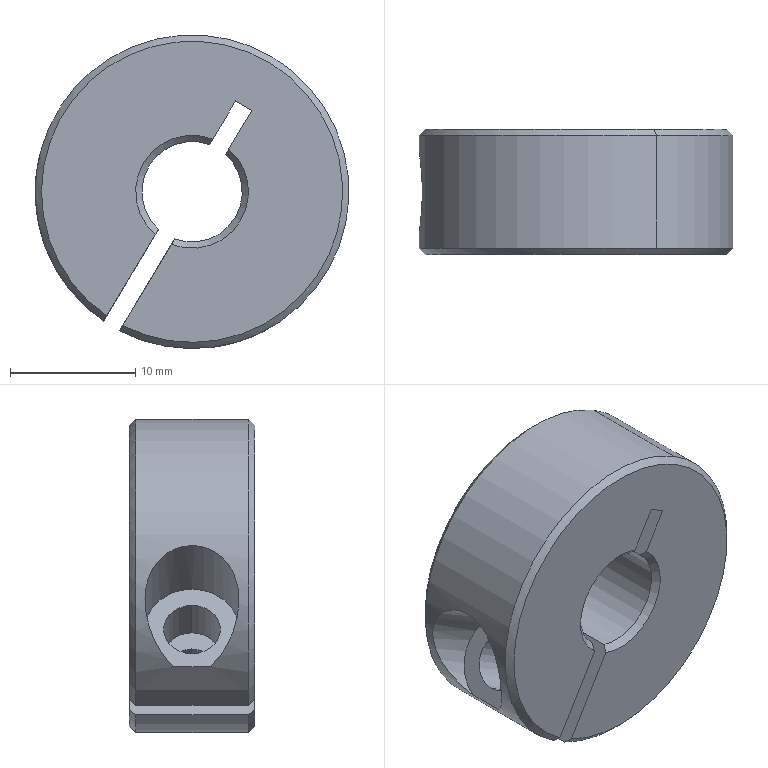Component | SolidWorks | F12529-M1072-1 | 1 solid | 24 faces | box 25 x 10 x 25 mm | volume 3862 mm3 | cylinder 9 | plane 8 | cone 7 | commonest cylinder face diameters 3.3 x2 4.5 x2 25 x2 8 x2 7.5 x1
build123d program:
from build123d import *

# Parameters (mm, degrees)
SKETCH1_R           = 12.5
SKETCH1_R_2         = 4
BOSS_EXTRUDE1_DEPTH = 10
CHAMFER1_SIZE       = 0.5
SKETCH2_W           = 1.5
SKETCH2_H           = 21
CUT_EXTRUDE1_DEPTH  = 12
SKETCH5_R           = 3.75
CUT_EXTRUDE2_DEPTH  = 10
SKETCH6_R           = 2.25
CUT_EXTRUDE3_DEPTH  = 5
M4_TAPPED_HOLE1_D   = 3.3


with BuildPart() as part:
    # Sketch1 → Boss-Extrude1 (new body)
    with BuildSketch(Plane(origin=(0, 0, 0), x_dir=(1, 0, 0), z_dir=(0, 1, 0))):
        with Locations(Location((0, 0, 0), (0, 0, 270))):
            Circle(SKETCH1_R)
        with Locations(Location((0, 0, 0), (0, 0, 270))):
            Circle(SKETCH1_R_2, mode=Mode.SUBTRACT)
    extrude(amount=BOSS_EXTRUDE1_DEPTH)

    # Chamfer1
    chamfer1_edges = [part.edges().sort_by_distance(p)[0] for p in [
        (0, 0, -12.5),
        (0, 10, -12.5),
        (0, 0, -4),
        (0, 10, -4),
    ]]
    chamfer(chamfer1_edges, length=CHAMFER1_SIZE)

    # Sketch2 → Cut-Extrude1 (cut)
    with BuildSketch(Plane(origin=(0, 10, 0), x_dir=(1, 0, 0), z_dir=(0, 1, 0))):
        with Locations((0, -2.5)):
            Rectangle(SKETCH2_W, SKETCH2_H)
    extrude(amount=-CUT_EXTRUDE1_DEPTH, mode=Mode.SUBTRACT)

    # Sketch5 → Cut-Extrude2 (cut)
    with BuildSketch(Plane(origin=(5, 0, 0), x_dir=(0, 0, -1), z_dir=(1, 0, 0))):
        with Locations((-8, 5)):
            Circle(SKETCH5_R)
    extrude(amount=CUT_EXTRUDE2_DEPTH, mode=Mode.SUBTRACT)

    # Sketch6 → Cut-Extrude3 (cut)
    with BuildSketch(Plane(origin=(5, 0, 0), x_dir=(0, 0, -1), z_dir=(1, 0, 0))):
        with Locations((-8, 5)):
            Circle(SKETCH6_R)
    extrude(amount=-CUT_EXTRUDE3_DEPTH, mode=Mode.SUBTRACT)

    # M4 Tapped Hole1 (through all)
    with Locations(Plane(origin=(-0.75, 0, 0), x_dir=(0, 0, -1), z_dir=(1, 0, 0))):
        with Locations((-8, 5)):
            Hole(M4_TAPPED_HOLE1_D / 2)


solid = part.part

# Placed as in the assembly
solid = solid.moved(Location((37.5, -20, 20), (179.999, -31.002, -179.999)))
STEP:
#1=COLOUR_RGB('',0.7922,0.8196,0.9333);
#2=FILL_AREA_STYLE_COLOUR('',#1);
#3=FILL_AREA_STYLE('',(#2));
#4=SURFACE_STYLE_FILL_AREA(#3);
#5=SURFACE_SIDE_STYLE('',(#4));
#6=SURFACE_STYLE_USAGE(.BOTH.,#5);
#7=PRESENTATION_STYLE_ASSIGNMENT((#6));
#8=CARTESIAN_POINT('',(1.549,-0.5906,0.3006));
#9=VERTEX_POINT('',#8);
#10=CARTESIAN_POINT('',(1.711,-0.5906,0.3548));
#11=VERTEX_POINT('',#10);
#12=CARTESIAN_POINT('',(1.549,-0.5906,0.3006));
#13=CARTESIAN_POINT('',(1.549,-0.5955,0.3006));
#14=CARTESIAN_POINT('',(1.55,-0.6005,0.3008));
#15=CARTESIAN_POINT('',(1.553,-0.6099,0.3013));
#16=CARTESIAN_POINT('',(1.555,-0.6143,0.3017));
#17=CARTESIAN_POINT('',(1.564,-0.6263,0.3031));
#18=CARTESIAN_POINT('',(1.572,-0.6329,0.3045));
#19=CARTESIAN_POINT('',(1.588,-0.6435,0.308));
#20=CARTESIAN_POINT('',(1.597,-0.6475,0.3102));
#21=CARTESIAN_POINT('',(1.615,-0.6533,0.3151));
#22=CARTESIAN_POINT('',(1.625,-0.655,0.318));
#23=CARTESIAN_POINT('',(1.643,-0.6558,0.3243));
#24=CARTESIAN_POINT('',(1.652,-0.655,0.3278));
#25=CARTESIAN_POINT('',(1.666,-0.6514,0.3332));
#26=CARTESIAN_POINT('',(1.67,-0.6498,0.335));
#27=CARTESIAN_POINT('',(1.678,-0.6458,0.3387));
#28=CARTESIAN_POINT('',(1.682,-0.6434,0.3405));
#29=CARTESIAN_POINT('',(1.694,-0.6349,0.3457));
#30=CARTESIAN_POINT('',(1.7,-0.6278,0.3489));
#31=CARTESIAN_POINT('',(1.706,-0.6147,0.3523));
#32=CARTESIAN_POINT('',(1.708,-0.6101,0.3532));
#33=CARTESIAN_POINT('',(1.71,-0.6006,0.3544));
#34=CARTESIAN_POINT('',(1.711,-0.5956,0.3548));
#35=CARTESIAN_POINT('',(1.711,-0.5906,0.3548));
#36=B_SPLINE_CURVE_WITH_KNOTS('',3,(#12,#13,#14,#15,#16,#17,#18,#19,#20,#21,#22,#23,#24,#25,#26,#27,#28,#29,#30,#31,#32,#33,#34,#35),.UNSPECIFIED.,.F.,.F.,(4,2,2,2,2,2,2,2,2,2,2,4),(0.006013,0.006389,0.006765,0.007517,0.008269,0.009021,0.009773,0.01015,0.01053,0.01128,0.01165,0.01203),.UNSPECIFIED.);
#37=EDGE_CURVE('',#9,#11,#36,.T.);
#38=ORIENTED_EDGE('',*,*,#37,.F.);
#39=CARTESIAN_POINT('',(1.306,-0.5906,0.4465));
#40=VERTEX_POINT('',#39);
#41=CARTESIAN_POINT('',(1.306,-0.5906,0.4465));
#42=DIRECTION('',(-0.8571,0.,0.5151));
#43=VECTOR('',#42,39.37);
#44=LINE('',#41,#43);
#45=EDGE_CURVE('',#9,#40,#44,.T.);
#46=ORIENTED_EDGE('',*,*,#45,.T.);
#47=CARTESIAN_POINT('',(1.373,-0.5906,0.5579));
#48=VERTEX_POINT('',#47);
#49=CARTESIAN_POINT('',(1.339,-0.5906,0.5022));
#50=DIRECTION('',(-0.8571,0.,0.5151));
#51=DIRECTION('',(0.5151,0.,0.8571));
#52=AXIS2_PLACEMENT_3D('',#49,#50,#51);
#53=CIRCLE('',#52,0.06496);
#54=EDGE_CURVE('',#40,#48,#53,.T.);
#55=ORIENTED_EDGE('',*,*,#54,.T.);
#56=CARTESIAN_POINT('',(1.373,-0.5906,0.5579));
#57=DIRECTION('',(-0.8571,0.,0.5151));
#58=VECTOR('',#57,39.37);
#59=LINE('',#56,#58);
#60=EDGE_CURVE('',#11,#48,#59,.T.);
#61=ORIENTED_EDGE('',*,*,#60,.F.);
#62=EDGE_LOOP('',(#38,#46,#55,#61));
#63=FACE_OUTER_BOUND('',#62,.T.);
#64=CARTESIAN_POINT('',(1.339,-0.5906,0.5022));
#65=DIRECTION('',(-0.8571,0.,0.5151));
#66=DIRECTION('',(0.5151,0.,0.8571));
#67=AXIS2_PLACEMENT_3D('',#64,#65,#66);
#68=CYLINDRICAL_SURFACE('',#67,0.06496);
#69=ADVANCED_FACE('',(#63),#68,.F.);
#70=CARTESIAN_POINT('',(1.243,-0.5906,0.4567));
#71=VERTEX_POINT('',#70);
#72=CARTESIAN_POINT('',(1.334,-0.5906,0.6086));
#73=VERTEX_POINT('',#72);
#74=CARTESIAN_POINT('',(1.289,-0.5906,0.5326));
#75=DIRECTION('',(-0.8571,0.,0.5151));
#76=DIRECTION('',(0.5151,0.,0.8571));
#77=AXIS2_PLACEMENT_3D('',#74,#75,#76);
#78=CIRCLE('',#77,0.08858);
#79=EDGE_CURVE('',#71,#73,#78,.T.);
#80=ORIENTED_EDGE('',*,*,#79,.F.);
#81=CARTESIAN_POINT('',(1.1,-0.5906,0.5429));
#82=VERTEX_POINT('',#81);
#83=CARTESIAN_POINT('',(1.269,-0.5906,0.4415));
#84=DIRECTION('',(-0.8571,0.,0.5151));
#85=VECTOR('',#84,39.37);
#86=LINE('',#83,#85);
#87=EDGE_CURVE('',#71,#82,#86,.T.);
#88=ORIENTED_EDGE('',*,*,#87,.T.);
#89=CARTESIAN_POINT('',(1.191,-0.5906,0.6948));
#90=VERTEX_POINT('',#89);
#91=CARTESIAN_POINT('',(1.145,-0.5906,0.6188));
#92=DIRECTION('',(-0.8571,0.,0.5151));
#93=DIRECTION('',(0.5151,0.,0.8571));
#94=AXIS2_PLACEMENT_3D('',#91,#92,#93);
#95=CIRCLE('',#94,0.08858);
#96=EDGE_CURVE('',#82,#90,#95,.T.);
#97=ORIENTED_EDGE('',*,*,#96,.T.);
#98=CARTESIAN_POINT('',(1.36,-0.5906,0.5934));
#99=DIRECTION('',(-0.8571,0.,0.5151));
#100=VECTOR('',#99,39.37);
#101=LINE('',#98,#100);
#102=EDGE_CURVE('',#73,#90,#101,.T.);
#103=ORIENTED_EDGE('',*,*,#102,.F.);
#104=EDGE_LOOP('',(#80,#88,#97,#103));
#105=FACE_OUTER_BOUND('',#104,.T.);
#106=CARTESIAN_POINT('',(1.314,-0.5906,0.5174));
#107=DIRECTION('',(-0.8571,0.,0.5151));
#108=DIRECTION('',(0.5151,0.,0.8571));
#109=AXIS2_PLACEMENT_3D('',#106,#107,#108);
#110=CYLINDRICAL_SURFACE('',#109,0.08858);
#111=ADVANCED_FACE('',(#105),#110,.F.);
#112=CARTESIAN_POINT('',(1.72,-0.3937,1.192));
#113=VERTEX_POINT('',#112);
#114=CARTESIAN_POINT('',(1.259,-0.3937,0.368));
#115=VERTEX_POINT('',#114);
#116=CARTESIAN_POINT('',(1.476,-0.3937,0.7874));
#117=DIRECTION('',(0.,1.,0.));
#118=DIRECTION('',(-0.5151,0.,-0.8571));
#119=AXIS2_PLACEMENT_3D('',#116,#117,#118);
#120=CIRCLE('',#119,0.4724);
#121=EDGE_CURVE('',#113,#115,#120,.T.);
#122=ORIENTED_EDGE('',*,*,#121,.F.);
#123=CARTESIAN_POINT('',(1.73,-0.4134,1.209));
#124=VERTEX_POINT('',#123);
#125=CARTESIAN_POINT('',(1.72,-0.3937,1.192));
#126=DIRECTION('',(0.3642,-0.7071,0.6061));
#127=VECTOR('',#126,39.37);
#128=LINE('',#125,#127);
#129=EDGE_CURVE('',#113,#124,#128,.T.);
#130=ORIENTED_EDGE('',*,*,#129,.T.);
#131=CARTESIAN_POINT('',(1.249,-0.4134,0.3511));
#132=VERTEX_POINT('',#131);
#133=CARTESIAN_POINT('',(1.476,-0.4134,0.7874));
#134=DIRECTION('',(0.,-1.,0.));
#135=DIRECTION('',(-0.5151,0.,-0.8571));
#136=AXIS2_PLACEMENT_3D('',#133,#134,#135);
#137=CIRCLE('',#136,0.4921);
#138=EDGE_CURVE('',#132,#124,#137,.T.);
#139=ORIENTED_EDGE('',*,*,#138,.F.);
#140=CARTESIAN_POINT('',(1.259,-0.3937,0.368));
#141=CARTESIAN_POINT('',(1.255,-0.4003,0.3624));
#142=CARTESIAN_POINT('',(1.252,-0.4068,0.3568));
#143=CARTESIAN_POINT('',(1.249,-0.4134,0.3511));
#144=B_SPLINE_CURVE_WITH_KNOTS('',3,(#140,#141,#142,#143),.UNSPECIFIED.,.F.,.F.,(4,4),(0.04478,0.04549),.UNSPECIFIED.);
#145=EDGE_CURVE('',#115,#132,#144,.T.);
#146=ORIENTED_EDGE('',*,*,#145,.F.);
#147=EDGE_LOOP('',(#122,#130,#139,#146));
#148=FACE_OUTER_BOUND('',#147,.T.);
#149=CARTESIAN_POINT('',(1.476,-0.3937,0.7874));
#150=DIRECTION('',(0.,-1.,0.));
#151=DIRECTION('',(0.5151,0.,0.8571));
#152=AXIS2_PLACEMENT_3D('',#149,#150,#151);
#153=CONICAL_SURFACE('',#152,0.4724,0.7854);
#154=ADVANCED_FACE('',(#148),#153,.T.);
#155=CARTESIAN_POINT('',(1.711,-0.5906,0.3548));
#156=CARTESIAN_POINT('',(1.711,-0.5855,0.3548));
#157=CARTESIAN_POINT('',(1.71,-0.5807,0.3545));
#158=CARTESIAN_POINT('',(1.708,-0.5711,0.3532));
#159=CARTESIAN_POINT('',(1.706,-0.5664,0.3523));
#160=CARTESIAN_POINT('',(1.702,-0.5579,0.3501));
#161=CARTESIAN_POINT('',(1.699,-0.5538,0.3487));
#162=CARTESIAN_POINT('',(1.693,-0.5466,0.3456));
#163=CARTESIAN_POINT('',(1.69,-0.5434,0.344));
#164=CARTESIAN_POINT('',(1.682,-0.5377,0.3405));
#165=CARTESIAN_POINT('',(1.679,-0.5353,0.3387));
#166=CARTESIAN_POINT('',(1.67,-0.5314,0.335));
#167=CARTESIAN_POINT('',(1.666,-0.5298,0.3332));
#168=CARTESIAN_POINT('',(1.653,-0.5262,0.3278));
#169=CARTESIAN_POINT('',(1.643,-0.5253,0.3243));
#170=CARTESIAN_POINT('',(1.624,-0.5261,0.318));
#171=CARTESIAN_POINT('',(1.615,-0.5278,0.3151));
#172=CARTESIAN_POINT('',(1.597,-0.5336,0.3101));
#173=CARTESIAN_POINT('',(1.588,-0.5376,0.308));
#174=CARTESIAN_POINT('',(1.576,-0.5456,0.3054));
#175=CARTESIAN_POINT('',(1.572,-0.5485,0.3046));
#176=CARTESIAN_POINT('',(1.565,-0.5551,0.3032));
#177=CARTESIAN_POINT('',(1.561,-0.5588,0.3026));
#178=CARTESIAN_POINT('',(1.555,-0.5669,0.3017));
#179=CARTESIAN_POINT('',(1.553,-0.5712,0.3013));
#180=CARTESIAN_POINT('',(1.55,-0.5806,0.3008));
#181=CARTESIAN_POINT('',(1.549,-0.5856,0.3006));
#182=CARTESIAN_POINT('',(1.549,-0.5906,0.3006));
#183=B_SPLINE_CURVE_WITH_KNOTS('',3,(#155,#156,#157,#158,#159,#160,#161,#162,#163,#164,#165,#166,#167,#168,#169,#170,#171,#172,#173,#174,#175,#176,#177,#178,#179,#180,#181,#182),.UNSPECIFIED.,.F.,.F.,(4,2,2,2,2,2,2,2,2,2,2,2,2,4),(0.,0.0003758,0.0007516,0.001127,0.001503,0.001879,0.002255,0.003006,0.003758,0.004509,0.004885,0.005261,0.005637,0.006013),.UNSPECIFIED.);
#184=EDGE_CURVE('',#11,#9,#183,.T.);
#185=ORIENTED_EDGE('',*,*,#184,.T.);
#186=ORIENTED_EDGE('',*,*,#37,.T.);
#187=EDGE_LOOP('',(#185,#186));
#188=FACE_BOUND('',#187,.T.);
#189=ORIENTED_EDGE('',*,*,#138,.T.);
#190=CARTESIAN_POINT('',(1.73,-0.7677,1.209));
#191=VERTEX_POINT('',#190);
#192=CARTESIAN_POINT('',(1.73,-0.3937,1.209));
#193=DIRECTION('',(0.,-1.,0.));
#194=VECTOR('',#193,39.37);
#195=LINE('',#192,#194);
#196=EDGE_CURVE('',#124,#191,#195,.T.);
#197=ORIENTED_EDGE('',*,*,#196,.T.);
#198=CARTESIAN_POINT('',(1.249,-0.7677,0.3511));
#199=VERTEX_POINT('',#198);
#200=CARTESIAN_POINT('',(1.476,-0.7677,0.7874));
#201=DIRECTION('',(0.,1.,0.));
#202=DIRECTION('',(-0.5151,0.,-0.8571));
#203=AXIS2_PLACEMENT_3D('',#200,#201,#202);
#204=CIRCLE('',#203,0.4921);
#205=EDGE_CURVE('',#191,#199,#204,.T.);
#206=ORIENTED_EDGE('',*,*,#205,.T.);
#207=CARTESIAN_POINT('',(1.249,-0.3937,0.3511));
#208=DIRECTION('',(0.,1.,0.));
#209=VECTOR('',#208,39.37);
#210=LINE('',#207,#209);
#211=EDGE_CURVE('',#199,#132,#210,.T.);
#212=ORIENTED_EDGE('',*,*,#211,.T.);
#213=EDGE_LOOP('',(#189,#197,#206,#212));
#214=FACE_OUTER_BOUND('',#213,.T.);
#215=CARTESIAN_POINT('',(1.476,-0.3937,0.7874));
#216=DIRECTION('',(0.,-1.,0.));
#217=DIRECTION('',(0.5151,0.,0.8571));
#218=AXIS2_PLACEMENT_3D('',#215,#216,#217);
#219=CYLINDRICAL_SURFACE('',#218,0.4921);
#220=ADVANCED_FACE('',(#188,#214),#219,.T.);
#221=CARTESIAN_POINT('',(1.422,-0.4134,0.6396));
#222=VERTEX_POINT('',#221);
#223=CARTESIAN_POINT('',(1.412,-0.3937,0.6225));
#224=VERTEX_POINT('',#223);
#225=CARTESIAN_POINT('',(1.422,-0.4134,0.6396));
#226=CARTESIAN_POINT('',(1.419,-0.4068,0.6339));
#227=CARTESIAN_POINT('',(1.415,-0.4003,0.6282));
#228=CARTESIAN_POINT('',(1.412,-0.3937,0.6225));
#229=B_SPLINE_CURVE_WITH_KNOTS('',3,(#225,#226,#227,#228),.UNSPECIFIED.,.F.,.F.,(4,4),(0.0187,0.01941),.UNSPECIFIED.);
#230=EDGE_CURVE('',#222,#224,#229,.T.);
#231=ORIENTED_EDGE('',*,*,#230,.T.);
#232=CARTESIAN_POINT('',(1.238,-0.3937,0.3335));
#233=DIRECTION('',(-0.5151,0.,-0.8571));
#234=VECTOR('',#233,39.37);
#235=LINE('',#232,#234);
#236=EDGE_CURVE('',#224,#115,#235,.T.);
#237=ORIENTED_EDGE('',*,*,#236,.T.);
#238=ORIENTED_EDGE('',*,*,#145,.T.);
#239=ORIENTED_EDGE('',*,*,#211,.F.);
#240=CARTESIAN_POINT('',(1.259,-0.7874,0.368));
#241=VERTEX_POINT('',#240);
#242=CARTESIAN_POINT('',(1.249,-0.7677,0.3511));
#243=CARTESIAN_POINT('',(1.252,-0.7743,0.3568));
#244=CARTESIAN_POINT('',(1.255,-0.7808,0.3624));
#245=CARTESIAN_POINT('',(1.259,-0.7874,0.368));
#246=B_SPLINE_CURVE_WITH_KNOTS('',3,(#242,#243,#244,#245),.UNSPECIFIED.,.F.,.F.,(4,4),(0.01741,0.01812),.UNSPECIFIED.);
#247=EDGE_CURVE('',#199,#241,#246,.T.);
#248=ORIENTED_EDGE('',*,*,#247,.T.);
#249=CARTESIAN_POINT('',(1.412,-0.7874,0.6225));
#250=VERTEX_POINT('',#249);
#251=CARTESIAN_POINT('',(1.502,-0.7874,0.7722));
#252=DIRECTION('',(-0.5151,0.,-0.8571));
#253=VECTOR('',#252,39.37);
#254=LINE('',#251,#253);
#255=EDGE_CURVE('',#250,#241,#254,.T.);
#256=ORIENTED_EDGE('',*,*,#255,.F.);
#257=CARTESIAN_POINT('',(1.422,-0.7677,0.6396));
#258=VERTEX_POINT('',#257);
#259=CARTESIAN_POINT('',(1.412,-0.7874,0.6225));
#260=CARTESIAN_POINT('',(1.415,-0.7808,0.6282));
#261=CARTESIAN_POINT('',(1.419,-0.7743,0.6339));
#262=CARTESIAN_POINT('',(1.422,-0.7677,0.6396));
#263=B_SPLINE_CURVE_WITH_KNOTS('',3,(#259,#260,#261,#262),.UNSPECIFIED.,.F.,.F.,(4,4),(0.007673,0.008386),.UNSPECIFIED.);
#264=EDGE_CURVE('',#250,#258,#263,.T.);
#265=ORIENTED_EDGE('',*,*,#264,.T.);
#266=CARTESIAN_POINT('',(1.422,-0.3937,0.6396));
#267=DIRECTION('',(0.,1.,0.));
#268=VECTOR('',#267,39.37);
#269=LINE('',#266,#268);
#270=EDGE_CURVE('',#258,#222,#269,.T.);
#271=ORIENTED_EDGE('',*,*,#270,.T.);
#272=EDGE_LOOP('',(#231,#237,#238,#239,#248,#256,#265,#271));
#273=FACE_OUTER_BOUND('',#272,.T.);
#274=CARTESIAN_POINT('',(1.339,-0.5906,0.5022));
#275=DIRECTION('',(-0.8571,0.,0.5151));
#276=DIRECTION('',(0.5151,0.,0.8571));
#277=AXIS2_PLACEMENT_3D('',#274,#275,#276);
#278=CIRCLE('',#277,0.06496);
#279=EDGE_CURVE('',#48,#40,#278,.T.);
#280=ORIENTED_EDGE('',*,*,#279,.F.);
#281=ORIENTED_EDGE('',*,*,#54,.F.);
#282=EDGE_LOOP('',(#280,#281));
#283=FACE_BOUND('',#282,.T.);
#284=CARTESIAN_POINT('',(1.238,-0.8661,0.3335));
#285=DIRECTION('',(0.8571,0.,-0.5151));
#286=DIRECTION('',(-0.5151,0.,-0.8571));
#287=AXIS2_PLACEMENT_3D('',#284,#285,#286);
#288=PLANE('',#287);
#289=ADVANCED_FACE('',(#273,#283),#288,.F.);
#290=ORIENTED_EDGE('',*,*,#196,.F.);
#291=CARTESIAN_POINT('',(1.198,-0.4134,0.3816));
#292=VERTEX_POINT('',#291);
#293=CARTESIAN_POINT('',(1.476,-0.4134,0.7874));
#294=DIRECTION('',(0.,-1.,0.));
#295=DIRECTION('',(-0.5151,0.,-0.8571));
#296=AXIS2_PLACEMENT_3D('',#293,#294,#295);
#297=CIRCLE('',#296,0.4921);
#298=EDGE_CURVE('',#124,#292,#297,.T.);
#299=ORIENTED_EDGE('',*,*,#298,.T.);
#300=CARTESIAN_POINT('',(1.198,-0.7677,0.3816));
#301=VERTEX_POINT('',#300);
#302=CARTESIAN_POINT('',(1.198,-0.3937,0.3816));
#303=DIRECTION('',(0.,-1.,0.));
#304=VECTOR('',#303,39.37);
#305=LINE('',#302,#304);
#306=EDGE_CURVE('',#292,#301,#305,.T.);
#307=ORIENTED_EDGE('',*,*,#306,.T.);
#308=CARTESIAN_POINT('',(1.476,-0.7677,0.7874));
#309=DIRECTION('',(0.,1.,0.));
#310=DIRECTION('',(-0.5151,0.,-0.8571));
#311=AXIS2_PLACEMENT_3D('',#308,#309,#310);
#312=CIRCLE('',#311,0.4921);
#313=EDGE_CURVE('',#301,#191,#312,.T.);
#314=ORIENTED_EDGE('',*,*,#313,.T.);
#315=EDGE_LOOP('',(#290,#299,#307,#314));
#316=FACE_OUTER_BOUND('',#315,.T.);
#317=CARTESIAN_POINT('',(1.075,-0.6478,0.5022));
#318=VERTEX_POINT('',#317);
#319=CARTESIAN_POINT('',(1.075,-0.5333,0.5022));
#320=VERTEX_POINT('',#319);
#321=CARTESIAN_POINT('',(1.075,-0.6478,0.5022));
#322=CARTESIAN_POINT('',(1.071,-0.6551,0.5084));
#323=CARTESIAN_POINT('',(1.066,-0.6617,0.5152));
#324=CARTESIAN_POINT('',(1.057,-0.6739,0.5295));
#325=CARTESIAN_POINT('',(1.053,-0.6796,0.537));
#326=CARTESIAN_POINT('',(1.044,-0.6903,0.5527));
#327=CARTESIAN_POINT('',(1.039,-0.6953,0.5609));
#328=CARTESIAN_POINT('',(1.031,-0.7045,0.5777));
#329=CARTESIAN_POINT('',(1.027,-0.7087,0.5864));
#330=CARTESIAN_POINT('',(1.016,-0.7203,0.613));
#331=CARTESIAN_POINT('',(1.009,-0.7266,0.6317));
#332=CARTESIAN_POINT('',(0.9977,-0.7356,0.6713));
#333=CARTESIAN_POINT('',(0.9932,-0.7382,0.6915));
#334=CARTESIAN_POINT('',(0.9884,-0.7382,0.7226));
#335=CARTESIAN_POINT('',(0.9871,-0.7375,0.7332));
#336=CARTESIAN_POINT('',(0.9853,-0.7347,0.7538));
#337=CARTESIAN_POINT('',(0.9847,-0.7325,0.764));
#338=CARTESIAN_POINT('',(0.9842,-0.7264,0.7841));
#339=CARTESIAN_POINT('',(0.9842,-0.7224,0.794));
#340=CARTESIAN_POINT('',(0.9848,-0.7128,0.8125));
#341=CARTESIAN_POINT('',(0.9853,-0.7072,0.8212));
#342=CARTESIAN_POINT('',(0.9867,-0.6941,0.8375));
#343=CARTESIAN_POINT('',(0.9876,-0.6865,0.8451));
#344=CARTESIAN_POINT('',(0.9893,-0.6703,0.8581));
#345=CARTESIAN_POINT('',(0.9902,-0.6615,0.8637));
#346=CARTESIAN_POINT('',(0.9917,-0.6424,0.8729));
#347=CARTESIAN_POINT('',(0.9924,-0.6325,0.8764));
#348=CARTESIAN_POINT('',(0.9933,-0.6121,0.8811));
#349=CARTESIAN_POINT('',(0.9935,-0.6014,0.8823));
#350=CARTESIAN_POINT('',(0.9935,-0.5805,0.8824));
#351=CARTESIAN_POINT('',(0.9933,-0.57,0.8813));
#352=CARTESIAN_POINT('',(0.9924,-0.5493,0.8766));
#353=CARTESIAN_POINT('',(0.9918,-0.5394,0.8732));
#354=CARTESIAN_POINT('',(0.9903,-0.5205,0.8642));
#355=CARTESIAN_POINT('',(0.9894,-0.5115,0.8585));
#356=CARTESIAN_POINT('',(0.9877,-0.4951,0.8456));
#357=CARTESIAN_POINT('',(0.9868,-0.4876,0.8382));
#358=CARTESIAN_POINT('',(0.9854,-0.4743,0.8218));
#359=CARTESIAN_POINT('',(0.9848,-0.4685,0.813));
#360=CARTESIAN_POINT('',(0.9842,-0.4589,0.7943));
#361=CARTESIAN_POINT('',(0.9842,-0.4549,0.7844));
#362=CARTESIAN_POINT('',(0.9847,-0.4487,0.7643));
#363=CARTESIAN_POINT('',(0.9853,-0.4465,0.7541));
#364=CARTESIAN_POINT('',(0.9871,-0.4436,0.7333));
#365=CARTESIAN_POINT('',(0.9884,-0.4429,0.7228));
#366=CARTESIAN_POINT('',(0.9916,-0.4429,0.7021));
#367=CARTESIAN_POINT('',(0.9935,-0.4435,0.6919));
#368=CARTESIAN_POINT('',(0.998,-0.446,0.6716));
#369=CARTESIAN_POINT('',(1.001,-0.4477,0.6614));
#370=CARTESIAN_POINT('',(1.009,-0.4545,0.6319));
#371=CARTESIAN_POINT('',(1.016,-0.4607,0.6132));
#372=CARTESIAN_POINT('',(1.031,-0.4763,0.5775));
#373=CARTESIAN_POINT('',(1.039,-0.4856,0.5604));
#374=CARTESIAN_POINT('',(1.053,-0.5015,0.5369));
#375=CARTESIAN_POINT('',(1.057,-0.5072,0.5295));
#376=CARTESIAN_POINT('',(1.066,-0.5194,0.5152));
#377=CARTESIAN_POINT('',(1.071,-0.526,0.5085));
#378=CARTESIAN_POINT('',(1.075,-0.5333,0.5022));
#379=B_SPLINE_CURVE_WITH_KNOTS('',3,(#321,#322,#323,#324,#325,#326,#327,#328,#329,#330,#331,#332,#333,#334,#335,#336,#337,#338,#339,#340,#341,#342,#343,#344,#345,#346,#347,#348,#349,#350,#351,#352,#353,#354,#355,#356,#357,#358,#359,#360,#361,#362,#363,#364,#365,#366,#367,#368,#369,#370,#371,#372,#373,#374,#375,#376,#377,#378),.UNSPECIFIED.,.F.,.F.,(4,2,2,2,2,2,2,2,2,2,2,2,2,2,2,2,2,2,2,2,2,2,2,2,2,2,2,2,4),(0.,0.0007962,0.001592,0.002389,0.003185,0.004777,0.00637,0.007166,0.007962,0.008759,0.009555,0.01035,0.01115,0.01194,0.01274,0.01354,0.01433,0.01513,0.01592,0.01672,0.01752,0.01831,0.01911,0.01991,0.0207,0.02229,0.02389,0.02468,0.02548),.UNSPECIFIED.);
#380=EDGE_CURVE('',#318,#320,#379,.T.);
#381=ORIENTED_EDGE('',*,*,#380,.F.);
#382=CARTESIAN_POINT('',(1.075,-0.3937,0.5022));
#383=DIRECTION('',(0.,-1.,0.));
#384=VECTOR('',#383,39.37);
#385=LINE('',#382,#384);
#386=EDGE_CURVE('',#320,#318,#385,.T.);
#387=ORIENTED_EDGE('',*,*,#386,.F.);
#388=EDGE_LOOP('',(#381,#387));
#389=FACE_BOUND('',#388,.T.);
#390=CARTESIAN_POINT('',(1.476,-0.3937,0.7874));
#391=DIRECTION('',(0.,-1.,0.));
#392=DIRECTION('',(0.5151,0.,0.8571));
#393=AXIS2_PLACEMENT_3D('',#390,#391,#392);
#394=CYLINDRICAL_SURFACE('',#393,0.4921);
#395=ADVANCED_FACE('',(#316,#389),#394,.T.);
#396=CARTESIAN_POINT('',(1.581,-0.4134,0.9048));
#397=VERTEX_POINT('',#396);
#398=CARTESIAN_POINT('',(1.581,-0.7677,0.9048));
#399=VERTEX_POINT('',#398);
#400=CARTESIAN_POINT('',(1.581,-0.3937,0.9048));
#401=DIRECTION('',(0.,-1.,0.));
#402=VECTOR('',#401,39.37);
#403=LINE('',#400,#402);
#404=EDGE_CURVE('',#397,#399,#403,.T.);
#405=ORIENTED_EDGE('',*,*,#404,.F.);
#406=CARTESIAN_POINT('',(1.476,-0.4134,0.7874));
#407=DIRECTION('',(0.,1.,0.));
#408=DIRECTION('',(-0.5151,0.,-0.8571));
#409=AXIS2_PLACEMENT_3D('',#406,#407,#408);
#410=CIRCLE('',#409,0.1575);
#411=EDGE_CURVE('',#397,#222,#410,.T.);
#412=ORIENTED_EDGE('',*,*,#411,.T.);
#413=ORIENTED_EDGE('',*,*,#270,.F.);
#414=CARTESIAN_POINT('',(1.476,-0.7677,0.7874));
#415=DIRECTION('',(0.,-1.,0.));
#416=DIRECTION('',(-0.5151,0.,-0.8571));
#417=AXIS2_PLACEMENT_3D('',#414,#415,#416);
#418=CIRCLE('',#417,0.1575);
#419=EDGE_CURVE('',#258,#399,#418,.T.);
#420=ORIENTED_EDGE('',*,*,#419,.T.);
#421=EDGE_LOOP('',(#405,#412,#413,#420));
#422=FACE_OUTER_BOUND('',#421,.T.);
#423=CARTESIAN_POINT('',(1.476,-0.3937,0.7874));
#424=DIRECTION('',(0.,-1.,0.));
#425=DIRECTION('',(0.5151,0.,0.8571));
#426=AXIS2_PLACEMENT_3D('',#423,#424,#425);
#427=CYLINDRICAL_SURFACE('',#426,0.1575);
#428=ADVANCED_FACE('',(#422),#427,.F.);
#429=ORIENTED_EDGE('',*,*,#264,.F.);
#430=CARTESIAN_POINT('',(1.592,-0.7874,0.9219));
#431=VERTEX_POINT('',#430);
#432=CARTESIAN_POINT('',(1.476,-0.7874,0.7874));
#433=DIRECTION('',(0.,1.,0.));
#434=DIRECTION('',(-0.5151,0.,-0.8571));
#435=AXIS2_PLACEMENT_3D('',#432,#433,#434);
#436=CIRCLE('',#435,0.1772);
#437=EDGE_CURVE('',#431,#250,#436,.T.);
#438=ORIENTED_EDGE('',*,*,#437,.F.);
#439=CARTESIAN_POINT('',(1.581,-0.7677,0.9048));
#440=CARTESIAN_POINT('',(1.585,-0.7743,0.9105));
#441=CARTESIAN_POINT('',(1.588,-0.7808,0.9162));
#442=CARTESIAN_POINT('',(1.592,-0.7874,0.9219));
#443=B_SPLINE_CURVE_WITH_KNOTS('',3,(#439,#440,#441,#442),.UNSPECIFIED.,.F.,.F.,(4,4),(0.0187,0.01941),.UNSPECIFIED.);
#444=EDGE_CURVE('',#399,#431,#443,.T.);
#445=ORIENTED_EDGE('',*,*,#444,.F.);
#446=ORIENTED_EDGE('',*,*,#419,.F.);
#447=EDGE_LOOP('',(#429,#438,#445,#446));
#448=FACE_OUTER_BOUND('',#447,.T.);
#449=CARTESIAN_POINT('',(1.476,-0.7874,0.7874));
#450=DIRECTION('',(0.,-1.,0.));
#451=DIRECTION('',(0.5151,0.,0.8571));
#452=AXIS2_PLACEMENT_3D('',#449,#450,#451);
#453=CONICAL_SURFACE('',#452,0.1772,0.7854);
#454=ADVANCED_FACE('',(#448),#453,.F.);
#455=CARTESIAN_POINT('',(1.592,-0.3937,0.9219));
#456=VERTEX_POINT('',#455);
#457=CARTESIAN_POINT('',(1.592,-0.3937,0.9219));
#458=CARTESIAN_POINT('',(1.588,-0.4003,0.9162));
#459=CARTESIAN_POINT('',(1.585,-0.4068,0.9105));
#460=CARTESIAN_POINT('',(1.581,-0.4134,0.9048));
#461=B_SPLINE_CURVE_WITH_KNOTS('',3,(#457,#458,#459,#460),.UNSPECIFIED.,.F.,.F.,(4,4),(0.007673,0.008386),.UNSPECIFIED.);
#462=EDGE_CURVE('',#456,#397,#461,.T.);
#463=ORIENTED_EDGE('',*,*,#462,.F.);
#464=CARTESIAN_POINT('',(1.476,-0.3937,0.7874));
#465=DIRECTION('',(0.,-1.,0.));
#466=DIRECTION('',(-0.5151,0.,-0.8571));
#467=AXIS2_PLACEMENT_3D('',#464,#465,#466);
#468=CIRCLE('',#467,0.1772);
#469=EDGE_CURVE('',#224,#456,#468,.T.);
#470=ORIENTED_EDGE('',*,*,#469,.F.);
#471=ORIENTED_EDGE('',*,*,#230,.F.);
#472=ORIENTED_EDGE('',*,*,#411,.F.);
#473=EDGE_LOOP('',(#463,#470,#471,#472));
#474=FACE_OUTER_BOUND('',#473,.T.);
#475=CARTESIAN_POINT('',(1.476,-0.4134,0.7874));
#476=DIRECTION('',(0.,1.,0.));
#477=DIRECTION('',(-0.5151,0.,-0.8571));
#478=AXIS2_PLACEMENT_3D('',#475,#476,#477);
#479=CONICAL_SURFACE('',#478,0.1575,0.7854);
#480=ADVANCED_FACE('',(#474),#479,.F.);
#481=ORIENTED_EDGE('',*,*,#236,.F.);
#482=ORIENTED_EDGE('',*,*,#469,.T.);
#483=CARTESIAN_POINT('',(1.664,-0.3937,1.042));
#484=VERTEX_POINT('',#483);
#485=CARTESIAN_POINT('',(1.238,-0.3937,0.3335));
#486=DIRECTION('',(-0.5151,0.,-0.8571));
#487=VECTOR('',#486,39.37);
#488=LINE('',#485,#487);
#489=EDGE_CURVE('',#484,#456,#488,.T.);
#490=ORIENTED_EDGE('',*,*,#489,.F.);
#491=CARTESIAN_POINT('',(1.613,-0.3937,1.073));
#492=VERTEX_POINT('',#491);
#493=CARTESIAN_POINT('',(1.664,-0.3937,1.042));
#494=DIRECTION('',(0.8571,0.,-0.5151));
#495=VECTOR('',#494,39.37);
#496=LINE('',#493,#495);
#497=EDGE_CURVE('',#492,#484,#496,.T.);
#498=ORIENTED_EDGE('',*,*,#497,.F.);
#499=CARTESIAN_POINT('',(1.541,-0.3937,0.9523));
#500=VERTEX_POINT('',#499);
#501=CARTESIAN_POINT('',(1.187,-0.3937,0.3639));
#502=DIRECTION('',(0.5151,0.,0.8571));
#503=VECTOR('',#502,39.37);
#504=LINE('',#501,#503);
#505=EDGE_CURVE('',#500,#492,#504,.T.);
#506=ORIENTED_EDGE('',*,*,#505,.F.);
#507=CARTESIAN_POINT('',(1.361,-0.3937,0.6529));
#508=VERTEX_POINT('',#507);
#509=CARTESIAN_POINT('',(1.476,-0.3937,0.7874));
#510=DIRECTION('',(0.,-1.,0.));
#511=DIRECTION('',(-0.5151,0.,-0.8571));
#512=AXIS2_PLACEMENT_3D('',#509,#510,#511);
#513=CIRCLE('',#512,0.1772);
#514=EDGE_CURVE('',#500,#508,#513,.T.);
#515=ORIENTED_EDGE('',*,*,#514,.T.);
#516=CARTESIAN_POINT('',(1.208,-0.3937,0.3985));
#517=VERTEX_POINT('',#516);
#518=CARTESIAN_POINT('',(1.187,-0.3937,0.3639));
#519=DIRECTION('',(0.5151,0.,0.8571));
#520=VECTOR('',#519,39.37);
#521=LINE('',#518,#520);
#522=EDGE_CURVE('',#517,#508,#521,.T.);
#523=ORIENTED_EDGE('',*,*,#522,.F.);
#524=CARTESIAN_POINT('',(1.476,-0.3937,0.7874));
#525=DIRECTION('',(0.,1.,0.));
#526=DIRECTION('',(-0.5151,0.,-0.8571));
#527=AXIS2_PLACEMENT_3D('',#524,#525,#526);
#528=CIRCLE('',#527,0.4724);
#529=EDGE_CURVE('',#517,#113,#528,.T.);
#530=ORIENTED_EDGE('',*,*,#529,.T.);
#531=ORIENTED_EDGE('',*,*,#121,.T.);
#532=EDGE_LOOP('',(#481,#482,#490,#498,#506,#515,#523,#530,#531));
#533=FACE_OUTER_BOUND('',#532,.T.);
#534=CARTESIAN_POINT('',(1.476,-0.3937,0.7874));
#535=DIRECTION('',(0.,1.,0.));
#536=DIRECTION('',(-0.5151,0.,-0.8571));
#537=AXIS2_PLACEMENT_3D('',#534,#535,#536);
#538=PLANE('',#537);
#539=ADVANCED_FACE('',(#533),#538,.T.);
#540=ORIENTED_EDGE('',*,*,#437,.T.);
#541=ORIENTED_EDGE('',*,*,#255,.T.);
#542=CARTESIAN_POINT('',(1.208,-0.7874,0.3985));
#543=VERTEX_POINT('',#542);
#544=CARTESIAN_POINT('',(1.476,-0.7874,0.7874));
#545=DIRECTION('',(0.,-1.,0.));
#546=DIRECTION('',(-0.5151,0.,-0.8571));
#547=AXIS2_PLACEMENT_3D('',#544,#545,#546);
#548=CIRCLE('',#547,0.4724);
#549=EDGE_CURVE('',#241,#543,#548,.T.);
#550=ORIENTED_EDGE('',*,*,#549,.T.);
#551=CARTESIAN_POINT('',(1.361,-0.7874,0.6529));
#552=VERTEX_POINT('',#551);
#553=CARTESIAN_POINT('',(1.451,-0.7874,0.8026));
#554=DIRECTION('',(0.5151,0.,0.8571));
#555=VECTOR('',#554,39.37);
#556=LINE('',#553,#555);
#557=EDGE_CURVE('',#543,#552,#556,.T.);
#558=ORIENTED_EDGE('',*,*,#557,.T.);
#559=CARTESIAN_POINT('',(1.541,-0.7874,0.9523));
#560=VERTEX_POINT('',#559);
#561=CARTESIAN_POINT('',(1.476,-0.7874,0.7874));
#562=DIRECTION('',(0.,1.,0.));
#563=DIRECTION('',(-0.5151,0.,-0.8571));
#564=AXIS2_PLACEMENT_3D('',#561,#562,#563);
#565=CIRCLE('',#564,0.1772);
#566=EDGE_CURVE('',#552,#560,#565,.T.);
#567=ORIENTED_EDGE('',*,*,#566,.T.);
#568=CARTESIAN_POINT('',(1.613,-0.7874,1.073));
#569=VERTEX_POINT('',#568);
#570=CARTESIAN_POINT('',(1.451,-0.7874,0.8026));
#571=DIRECTION('',(0.5151,0.,0.8571));
#572=VECTOR('',#571,39.37);
#573=LINE('',#570,#572);
#574=EDGE_CURVE('',#560,#569,#573,.T.);
#575=ORIENTED_EDGE('',*,*,#574,.T.);
#576=CARTESIAN_POINT('',(1.664,-0.7874,1.042));
#577=VERTEX_POINT('',#576);
#578=CARTESIAN_POINT('',(1.639,-0.7874,1.057));
#579=DIRECTION('',(0.8571,0.,-0.5151));
#580=VECTOR('',#579,39.37);
#581=LINE('',#578,#580);
#582=EDGE_CURVE('',#569,#577,#581,.T.);
#583=ORIENTED_EDGE('',*,*,#582,.T.);
#584=CARTESIAN_POINT('',(1.502,-0.7874,0.7722));
#585=DIRECTION('',(-0.5151,0.,-0.8571));
#586=VECTOR('',#585,39.37);
#587=LINE('',#584,#586);
#588=EDGE_CURVE('',#577,#431,#587,.T.);
#589=ORIENTED_EDGE('',*,*,#588,.T.);
#590=EDGE_LOOP('',(#540,#541,#550,#558,#567,#575,#583,#589));
#591=FACE_OUTER_BOUND('',#590,.T.);
#592=CARTESIAN_POINT('',(1.476,-0.7874,0.7874));
#593=DIRECTION('',(0.,1.,0.));
#594=DIRECTION('',(-0.5151,0.,-0.8571));
#595=AXIS2_PLACEMENT_3D('',#592,#593,#594);
#596=PLANE('',#595);
#597=ADVANCED_FACE('',(#591),#596,.F.);
#598=CARTESIAN_POINT('',(1.371,-0.4134,0.67));
#599=VERTEX_POINT('',#598);
#600=CARTESIAN_POINT('',(1.371,-0.7677,0.67));
#601=VERTEX_POINT('',#600);
#602=CARTESIAN_POINT('',(1.371,-0.3937,0.67));
#603=DIRECTION('',(0.,-1.,0.));
#604=VECTOR('',#603,39.37);
#605=LINE('',#602,#604);
#606=EDGE_CURVE('',#599,#601,#605,.T.);
#607=ORIENTED_EDGE('',*,*,#606,.F.);
#608=CARTESIAN_POINT('',(1.531,-0.4134,0.9352));
#609=VERTEX_POINT('',#608);
#610=CARTESIAN_POINT('',(1.476,-0.4134,0.7874));
#611=DIRECTION('',(0.,1.,0.));
#612=DIRECTION('',(-0.5151,0.,-0.8571));
#613=AXIS2_PLACEMENT_3D('',#610,#611,#612);
#614=CIRCLE('',#613,0.1575);
#615=EDGE_CURVE('',#599,#609,#614,.T.);
#616=ORIENTED_EDGE('',*,*,#615,.T.);
#617=CARTESIAN_POINT('',(1.531,-0.7677,0.9352));
#618=VERTEX_POINT('',#617);
#619=CARTESIAN_POINT('',(1.531,-0.3937,0.9352));
#620=DIRECTION('',(0.,1.,0.));
#621=VECTOR('',#620,39.37);
#622=LINE('',#619,#621);
#623=EDGE_CURVE('',#618,#609,#622,.T.);
#624=ORIENTED_EDGE('',*,*,#623,.F.);
#625=CARTESIAN_POINT('',(1.476,-0.7677,0.7874));
#626=DIRECTION('',(0.,-1.,0.));
#627=DIRECTION('',(-0.5151,0.,-0.8571));
#628=AXIS2_PLACEMENT_3D('',#625,#626,#627);
#629=CIRCLE('',#628,0.1575);
#630=EDGE_CURVE('',#618,#601,#629,.T.);
#631=ORIENTED_EDGE('',*,*,#630,.T.);
#632=EDGE_LOOP('',(#607,#616,#624,#631));
#633=FACE_OUTER_BOUND('',#632,.T.);
#634=CARTESIAN_POINT('',(1.476,-0.3937,0.7874));
#635=DIRECTION('',(0.,-1.,0.));
#636=DIRECTION('',(0.5151,0.,0.8571));
#637=AXIS2_PLACEMENT_3D('',#634,#635,#636);
#638=CYLINDRICAL_SURFACE('',#637,0.1575);
#639=ADVANCED_FACE('',(#633),#638,.F.);
#640=CARTESIAN_POINT('',(1.541,-0.7874,0.9523));
#641=CARTESIAN_POINT('',(1.538,-0.7808,0.9466));
#642=CARTESIAN_POINT('',(1.534,-0.7743,0.9409));
#643=CARTESIAN_POINT('',(1.531,-0.7677,0.9352));
#644=B_SPLINE_CURVE_WITH_KNOTS('',3,(#640,#641,#642,#643),.UNSPECIFIED.,.F.,.F.,(4,4),(0.007673,0.008386),.UNSPECIFIED.);
#645=EDGE_CURVE('',#560,#618,#644,.T.);
#646=ORIENTED_EDGE('',*,*,#645,.F.);
#647=ORIENTED_EDGE('',*,*,#566,.F.);
#648=CARTESIAN_POINT('',(1.371,-0.7677,0.67));
#649=CARTESIAN_POINT('',(1.368,-0.7743,0.6643));
#650=CARTESIAN_POINT('',(1.365,-0.7808,0.6586));
#651=CARTESIAN_POINT('',(1.361,-0.7874,0.6529));
#652=B_SPLINE_CURVE_WITH_KNOTS('',3,(#648,#649,#650,#651),.UNSPECIFIED.,.F.,.F.,(4,4),(0.0187,0.01941),.UNSPECIFIED.);
#653=EDGE_CURVE('',#601,#552,#652,.T.);
#654=ORIENTED_EDGE('',*,*,#653,.F.);
#655=ORIENTED_EDGE('',*,*,#630,.F.);
#656=EDGE_LOOP('',(#646,#647,#654,#655));
#657=FACE_OUTER_BOUND('',#656,.T.);
#658=CARTESIAN_POINT('',(1.476,-0.7874,0.7874));
#659=DIRECTION('',(0.,-1.,0.));
#660=DIRECTION('',(0.5151,0.,0.8571));
#661=AXIS2_PLACEMENT_3D('',#658,#659,#660);
#662=CONICAL_SURFACE('',#661,0.1772,0.7854);
#663=ADVANCED_FACE('',(#657),#662,.F.);
#664=ORIENTED_EDGE('',*,*,#247,.F.);
#665=ORIENTED_EDGE('',*,*,#205,.F.);
#666=ORIENTED_EDGE('',*,*,#313,.F.);
#667=CARTESIAN_POINT('',(1.208,-0.7874,0.3985));
#668=CARTESIAN_POINT('',(1.205,-0.7808,0.3928));
#669=CARTESIAN_POINT('',(1.201,-0.7743,0.3872));
#670=CARTESIAN_POINT('',(1.198,-0.7677,0.3816));
#671=B_SPLINE_CURVE_WITH_KNOTS('',3,(#667,#668,#669,#670),.UNSPECIFIED.,.F.,.F.,(4,4),(0.04478,0.04549),.UNSPECIFIED.);
#672=EDGE_CURVE('',#543,#301,#671,.T.);
#673=ORIENTED_EDGE('',*,*,#672,.F.);
#674=ORIENTED_EDGE('',*,*,#549,.F.);
#675=EDGE_LOOP('',(#664,#665,#666,#673,#674));
#676=FACE_OUTER_BOUND('',#675,.T.);
#677=CARTESIAN_POINT('',(1.476,-0.7677,0.7874));
#678=DIRECTION('',(0.,1.,0.));
#679=DIRECTION('',(-0.5151,0.,-0.8571));
#680=AXIS2_PLACEMENT_3D('',#677,#678,#679);
#681=CONICAL_SURFACE('',#680,0.4921,0.7854);
#682=ADVANCED_FACE('',(#676),#681,.T.);
#683=CARTESIAN_POINT('',(1.361,-0.3937,0.6529));
#684=CARTESIAN_POINT('',(1.365,-0.4003,0.6586));
#685=CARTESIAN_POINT('',(1.368,-0.4068,0.6643));
#686=CARTESIAN_POINT('',(1.371,-0.4134,0.67));
#687=B_SPLINE_CURVE_WITH_KNOTS('',3,(#683,#684,#685,#686),.UNSPECIFIED.,.F.,.F.,(4,4),(0.007673,0.008386),.UNSPECIFIED.);
#688=EDGE_CURVE('',#508,#599,#687,.T.);
#689=ORIENTED_EDGE('',*,*,#688,.F.);
#690=ORIENTED_EDGE('',*,*,#514,.F.);
#691=CARTESIAN_POINT('',(1.531,-0.4134,0.9352));
#692=CARTESIAN_POINT('',(1.534,-0.4068,0.9409));
#693=CARTESIAN_POINT('',(1.538,-0.4003,0.9466));
#694=CARTESIAN_POINT('',(1.541,-0.3937,0.9523));
#695=B_SPLINE_CURVE_WITH_KNOTS('',3,(#691,#692,#693,#694),.UNSPECIFIED.,.F.,.F.,(4,4),(0.0187,0.01941),.UNSPECIFIED.);
#696=EDGE_CURVE('',#609,#500,#695,.T.);
#697=ORIENTED_EDGE('',*,*,#696,.F.);
#698=ORIENTED_EDGE('',*,*,#615,.F.);
#699=EDGE_LOOP('',(#689,#690,#697,#698));
#700=FACE_OUTER_BOUND('',#699,.T.);
#701=CARTESIAN_POINT('',(1.476,-0.4134,0.7874));
#702=DIRECTION('',(0.,1.,0.));
#703=DIRECTION('',(-0.5151,0.,-0.8571));
#704=AXIS2_PLACEMENT_3D('',#701,#702,#703);
#705=CONICAL_SURFACE('',#704,0.1575,0.7854);
#706=ADVANCED_FACE('',(#700),#705,.F.);
#707=ORIENTED_EDGE('',*,*,#129,.F.);
#708=ORIENTED_EDGE('',*,*,#529,.F.);
#709=CARTESIAN_POINT('',(1.198,-0.4134,0.3816));
#710=CARTESIAN_POINT('',(1.201,-0.4068,0.3872));
#711=CARTESIAN_POINT('',(1.205,-0.4003,0.3928));
#712=CARTESIAN_POINT('',(1.208,-0.3937,0.3985));
#713=B_SPLINE_CURVE_WITH_KNOTS('',3,(#709,#710,#711,#712),.UNSPECIFIED.,.F.,.F.,(4,4),(0.01741,0.01812),.UNSPECIFIED.);
#714=EDGE_CURVE('',#292,#517,#713,.T.);
#715=ORIENTED_EDGE('',*,*,#714,.F.);
#716=ORIENTED_EDGE('',*,*,#298,.F.);
#717=EDGE_LOOP('',(#707,#708,#715,#716));
#718=FACE_OUTER_BOUND('',#717,.T.);
#719=CARTESIAN_POINT('',(1.476,-0.3937,0.7874));
#720=DIRECTION('',(0.,-1.,0.));
#721=DIRECTION('',(0.5151,0.,0.8571));
#722=AXIS2_PLACEMENT_3D('',#719,#720,#721);
#723=CONICAL_SURFACE('',#722,0.4724,0.7854);
#724=ADVANCED_FACE('',(#718),#723,.T.);
#725=CARTESIAN_POINT('',(1.289,-0.5906,0.5326));
#726=DIRECTION('',(-0.8571,0.,0.5151));
#727=DIRECTION('',(0.5151,0.,0.8571));
#728=AXIS2_PLACEMENT_3D('',#725,#726,#727);
#729=CIRCLE('',#728,0.08858);
#730=EDGE_CURVE('',#73,#71,#729,.T.);
#731=ORIENTED_EDGE('',*,*,#730,.T.);
#732=ORIENTED_EDGE('',*,*,#79,.T.);
#733=EDGE_LOOP('',(#731,#732));
#734=FACE_BOUND('',#733,.T.);
#735=ORIENTED_EDGE('',*,*,#688,.T.);
#736=ORIENTED_EDGE('',*,*,#606,.T.);
#737=ORIENTED_EDGE('',*,*,#653,.T.);
#738=ORIENTED_EDGE('',*,*,#557,.F.);
#739=ORIENTED_EDGE('',*,*,#672,.T.);
#740=ORIENTED_EDGE('',*,*,#306,.F.);
#741=ORIENTED_EDGE('',*,*,#714,.T.);
#742=ORIENTED_EDGE('',*,*,#522,.T.);
#743=EDGE_LOOP('',(#735,#736,#737,#738,#739,#740,#741,#742));
#744=FACE_OUTER_BOUND('',#743,.T.);
#745=CARTESIAN_POINT('',(1.187,-0.8661,0.3639));
#746=DIRECTION('',(-0.8571,0.,0.5151));
#747=DIRECTION('',(0.5151,0.,0.8571));
#748=AXIS2_PLACEMENT_3D('',#745,#746,#747);
#749=PLANE('',#748);
#750=ADVANCED_FACE('',(#734,#744),#749,.F.);
#751=CARTESIAN_POINT('',(1.613,-0.8661,1.073));
#752=DIRECTION('',(0.,1.,0.));
#753=VECTOR('',#752,39.37);
#754=LINE('',#751,#753);
#755=EDGE_CURVE('',#569,#492,#754,.T.);
#756=ORIENTED_EDGE('',*,*,#755,.T.);
#757=ORIENTED_EDGE('',*,*,#497,.T.);
#758=CARTESIAN_POINT('',(1.664,-0.8661,1.042));
#759=DIRECTION('',(0.,1.,0.));
#760=VECTOR('',#759,39.37);
#761=LINE('',#758,#760);
#762=EDGE_CURVE('',#577,#484,#761,.T.);
#763=ORIENTED_EDGE('',*,*,#762,.F.);
#764=ORIENTED_EDGE('',*,*,#582,.F.);
#765=EDGE_LOOP('',(#756,#757,#763,#764));
#766=FACE_OUTER_BOUND('',#765,.T.);
#767=CARTESIAN_POINT('',(1.664,-0.8661,1.042));
#768=DIRECTION('',(0.5151,0.,0.8571));
#769=DIRECTION('',(0.8571,0.,-0.5151));
#770=AXIS2_PLACEMENT_3D('',#767,#768,#769);
#771=PLANE('',#770);
#772=ADVANCED_FACE('',(#766),#771,.F.);
#773=ORIENTED_EDGE('',*,*,#762,.T.);
#774=ORIENTED_EDGE('',*,*,#489,.T.);
#775=ORIENTED_EDGE('',*,*,#462,.T.);
#776=ORIENTED_EDGE('',*,*,#404,.T.);
#777=ORIENTED_EDGE('',*,*,#444,.T.);
#778=ORIENTED_EDGE('',*,*,#588,.F.);
#779=EDGE_LOOP('',(#773,#774,#775,#776,#777,#778));
#780=FACE_OUTER_BOUND('',#779,.T.);
#781=CARTESIAN_POINT('',(1.238,-0.8661,0.3335));
#782=DIRECTION('',(0.8571,0.,-0.5151));
#783=DIRECTION('',(-0.5151,0.,-0.8571));
#784=AXIS2_PLACEMENT_3D('',#781,#782,#783);
#785=PLANE('',#784);
#786=ADVANCED_FACE('',(#780),#785,.F.);
#787=ORIENTED_EDGE('',*,*,#645,.T.);
#788=ORIENTED_EDGE('',*,*,#623,.T.);
#789=ORIENTED_EDGE('',*,*,#696,.T.);
#790=ORIENTED_EDGE('',*,*,#505,.T.);
#791=ORIENTED_EDGE('',*,*,#755,.F.);
#792=ORIENTED_EDGE('',*,*,#574,.F.);
#793=EDGE_LOOP('',(#787,#788,#789,#790,#791,#792));
#794=FACE_OUTER_BOUND('',#793,.T.);
#795=CARTESIAN_POINT('',(1.187,-0.8661,0.3639));
#796=DIRECTION('',(-0.8571,0.,0.5151));
#797=DIRECTION('',(0.5151,0.,0.8571));
#798=AXIS2_PLACEMENT_3D('',#795,#796,#797);
#799=PLANE('',#798);
#800=ADVANCED_FACE('',(#794),#799,.F.);
#801=ORIENTED_EDGE('',*,*,#380,.T.);
#802=CARTESIAN_POINT('',(1.145,-0.5906,0.6188));
#803=DIRECTION('',(-0.8571,0.,0.5151));
#804=DIRECTION('',(0.5151,0.,0.8571));
#805=AXIS2_PLACEMENT_3D('',#802,#803,#804);
#806=CIRCLE('',#805,0.1476);
#807=EDGE_CURVE('',#318,#320,#806,.T.);
#808=ORIENTED_EDGE('',*,*,#807,.F.);
#809=EDGE_LOOP('',(#801,#808));
#810=FACE_OUTER_BOUND('',#809,.T.);
#811=CARTESIAN_POINT('',(0.808,-0.5906,0.8216));
#812=DIRECTION('',(0.8571,0.,-0.5151));
#813=DIRECTION('',(-0.5151,0.,-0.8571));
#814=AXIS2_PLACEMENT_3D('',#811,#812,#813);
#815=CYLINDRICAL_SURFACE('',#814,0.1476);
#816=ADVANCED_FACE('',(#810),#815,.F.);
#817=CARTESIAN_POINT('',(1.145,-0.5906,0.6188));
#818=DIRECTION('',(-0.8571,0.,0.5151));
#819=DIRECTION('',(0.5151,0.,0.8571));
#820=AXIS2_PLACEMENT_3D('',#817,#818,#819);
#821=CIRCLE('',#820,0.08858);
#822=EDGE_CURVE('',#90,#82,#821,.T.);
#823=ORIENTED_EDGE('',*,*,#822,.F.);
#824=ORIENTED_EDGE('',*,*,#96,.F.);
#825=EDGE_LOOP('',(#823,#824));
#826=FACE_BOUND('',#825,.T.);
#827=ORIENTED_EDGE('',*,*,#386,.T.);
#828=ORIENTED_EDGE('',*,*,#807,.T.);
#829=EDGE_LOOP('',(#827,#828));
#830=FACE_OUTER_BOUND('',#829,.T.);
#831=CARTESIAN_POINT('',(1.145,-0.5906,0.6188));
#832=DIRECTION('',(-0.8571,0.,0.5151));
#833=DIRECTION('',(0.5151,0.,0.8571));
#834=AXIS2_PLACEMENT_3D('',#831,#832,#833);
#835=PLANE('',#834);
#836=ADVANCED_FACE('',(#826,#830),#835,.T.);
#837=ORIENTED_EDGE('',*,*,#87,.F.);
#838=ORIENTED_EDGE('',*,*,#730,.F.);
#839=ORIENTED_EDGE('',*,*,#102,.T.);
#840=ORIENTED_EDGE('',*,*,#822,.T.);
#841=EDGE_LOOP('',(#837,#838,#839,#840));
#842=FACE_OUTER_BOUND('',#841,.T.);
#843=CARTESIAN_POINT('',(1.314,-0.5906,0.5174));
#844=DIRECTION('',(-0.8571,0.,0.5151));
#845=DIRECTION('',(0.5151,0.,0.8571));
#846=AXIS2_PLACEMENT_3D('',#843,#844,#845);
#847=CYLINDRICAL_SURFACE('',#846,0.08858);
#848=ADVANCED_FACE('',(#842),#847,.F.);
#849=ORIENTED_EDGE('',*,*,#45,.F.);
#850=ORIENTED_EDGE('',*,*,#184,.F.);
#851=ORIENTED_EDGE('',*,*,#60,.T.);
#852=ORIENTED_EDGE('',*,*,#279,.T.);
#853=EDGE_LOOP('',(#849,#850,#851,#852));
#854=FACE_OUTER_BOUND('',#853,.T.);
#855=CARTESIAN_POINT('',(1.339,-0.5906,0.5022));
#856=DIRECTION('',(-0.8571,0.,0.5151));
#857=DIRECTION('',(0.5151,0.,0.8571));
#858=AXIS2_PLACEMENT_3D('',#855,#856,#857);
#859=CYLINDRICAL_SURFACE('',#858,0.06496);
#860=ADVANCED_FACE('',(#854),#859,.F.);
#861=CLOSED_SHELL('',(#69,#111,#154,#220,#289,#395,#428,#454,#480,#539,#597,#639,#663,#682,#706,#724,#750,#772,#786,#800,#816,#836,#848,#860));
#862=MANIFOLD_SOLID_BREP('',#861);
#863=STYLED_ITEM('',(#7),#862);
#864=(LENGTH_UNIT()NAMED_UNIT(*)SI_UNIT($,.METRE.));
#865=LENGTH_MEASURE_WITH_UNIT(LENGTH_MEASURE(0.0254),#864);
#866=DIMENSIONAL_EXPONENTS(1.,0.,0.,0.,0.,0.,0.);
#867=(CONVERSION_BASED_UNIT('',#865)LENGTH_UNIT()NAMED_UNIT(#866));
#868=UNCERTAINTY_MEASURE_WITH_UNIT(LENGTH_MEASURE(0.00001),#867,'','');
#869=(NAMED_UNIT(*)PLANE_ANGLE_UNIT()SI_UNIT($,.RADIAN.));
#870=(NAMED_UNIT(*)SI_UNIT($,.STERADIAN.)SOLID_ANGLE_UNIT());
#871=(GEOMETRIC_REPRESENTATION_CONTEXT(3)GLOBAL_UNCERTAINTY_ASSIGNED_CONTEXT((#868))GLOBAL_UNIT_ASSIGNED_CONTEXT((#867,#869,#870))REPRESENTATION_CONTEXT('',''));
#872=MECHANICAL_DESIGN_GEOMETRIC_PRESENTATION_REPRESENTATION('',(#863),#871);
#873=PRESENTATION_LAYER_ASSIGNMENT('','',(#863));
#874=CARTESIAN_POINT('',(0.,0.,0.));
#875=DIRECTION('',(0.,0.,1.));
#876=DIRECTION('',(1.,0.,0.));
#877=AXIS2_PLACEMENT_3D('',#874,#875,#876);
#878=(LENGTH_UNIT()NAMED_UNIT(*)SI_UNIT($,.METRE.));
#879=LENGTH_MEASURE_WITH_UNIT(LENGTH_MEASURE(0.0254),#878);
#880=DIMENSIONAL_EXPONENTS(1.,0.,0.,0.,0.,0.,0.);
#881=(CONVERSION_BASED_UNIT('',#879)LENGTH_UNIT()NAMED_UNIT(#880));
#882=UNCERTAINTY_MEASURE_WITH_UNIT(LENGTH_MEASURE(0.00001),#881,'','');
#883=(NAMED_UNIT(*)PLANE_ANGLE_UNIT()SI_UNIT($,.RADIAN.));
#884=(NAMED_UNIT(*)SI_UNIT($,.STERADIAN.)SOLID_ANGLE_UNIT());
#885=(GEOMETRIC_REPRESENTATION_CONTEXT(3)GLOBAL_UNCERTAINTY_ASSIGNED_CONTEXT((#882))GLOBAL_UNIT_ASSIGNED_CONTEXT((#881,#883,#884))REPRESENTATION_CONTEXT('',''));
#886=ADVANCED_BREP_SHAPE_REPRESENTATION('',(#862,#877),#885);